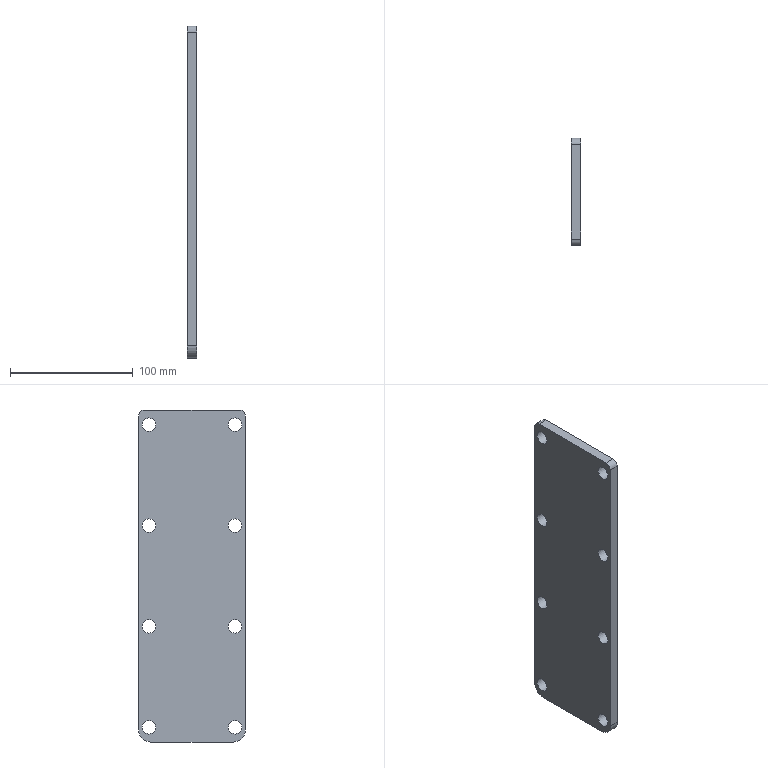Component | NX | HOUSING_COVER | 1 solid | 18 faces | volume 181409 mm3 | cylinder 12 | plane 6 | commonest cylinder face diameters 11 x8 10 x2 20 x2